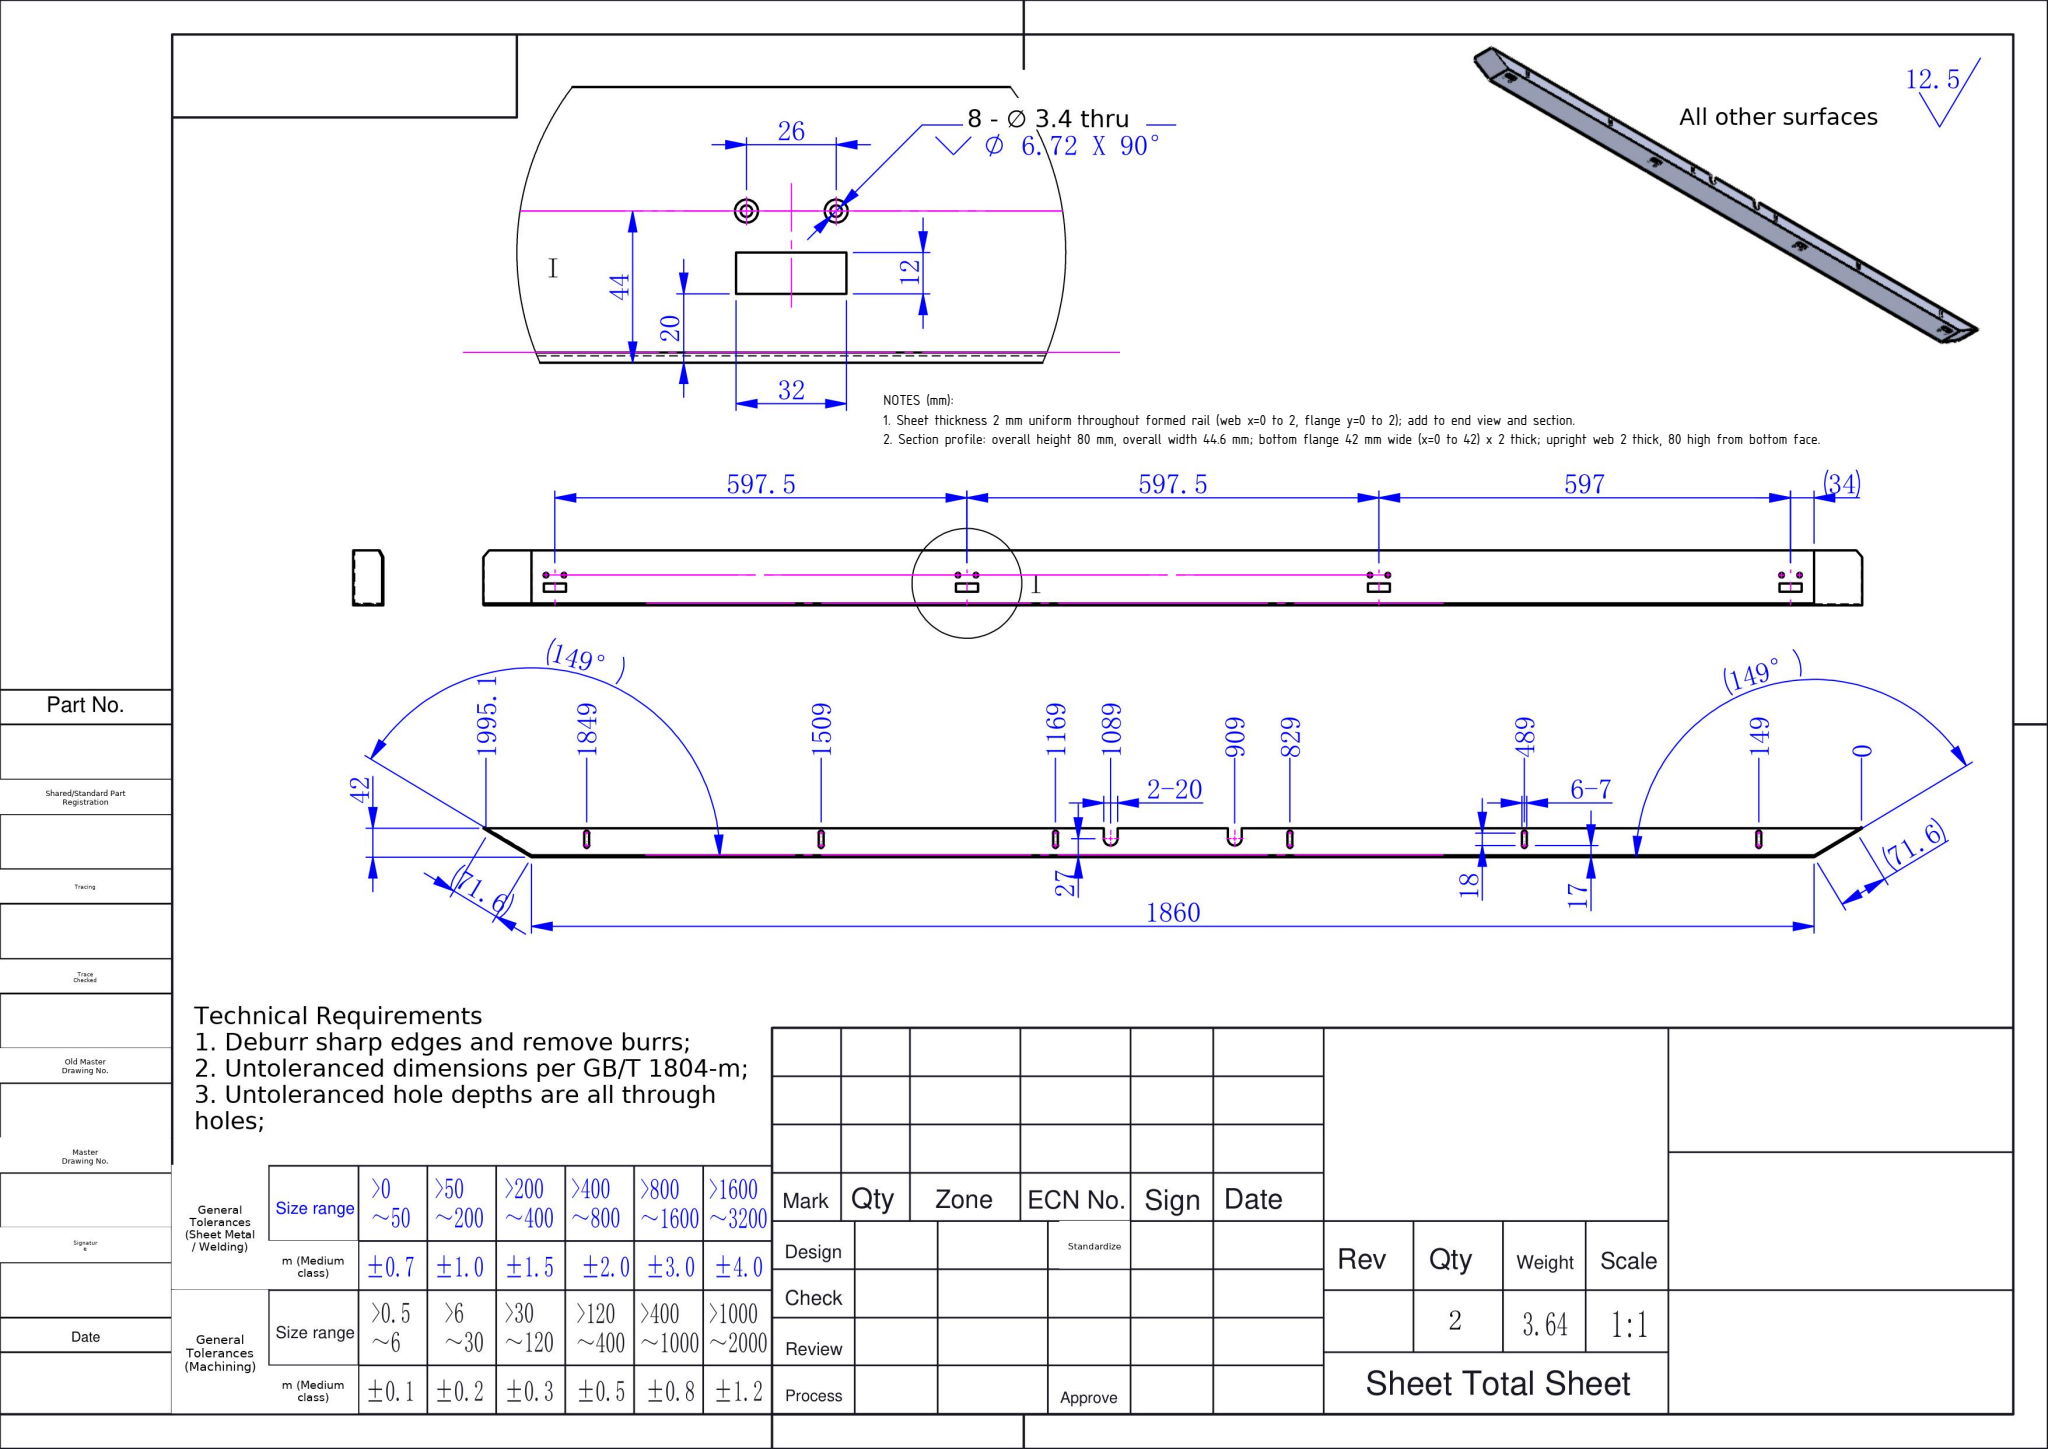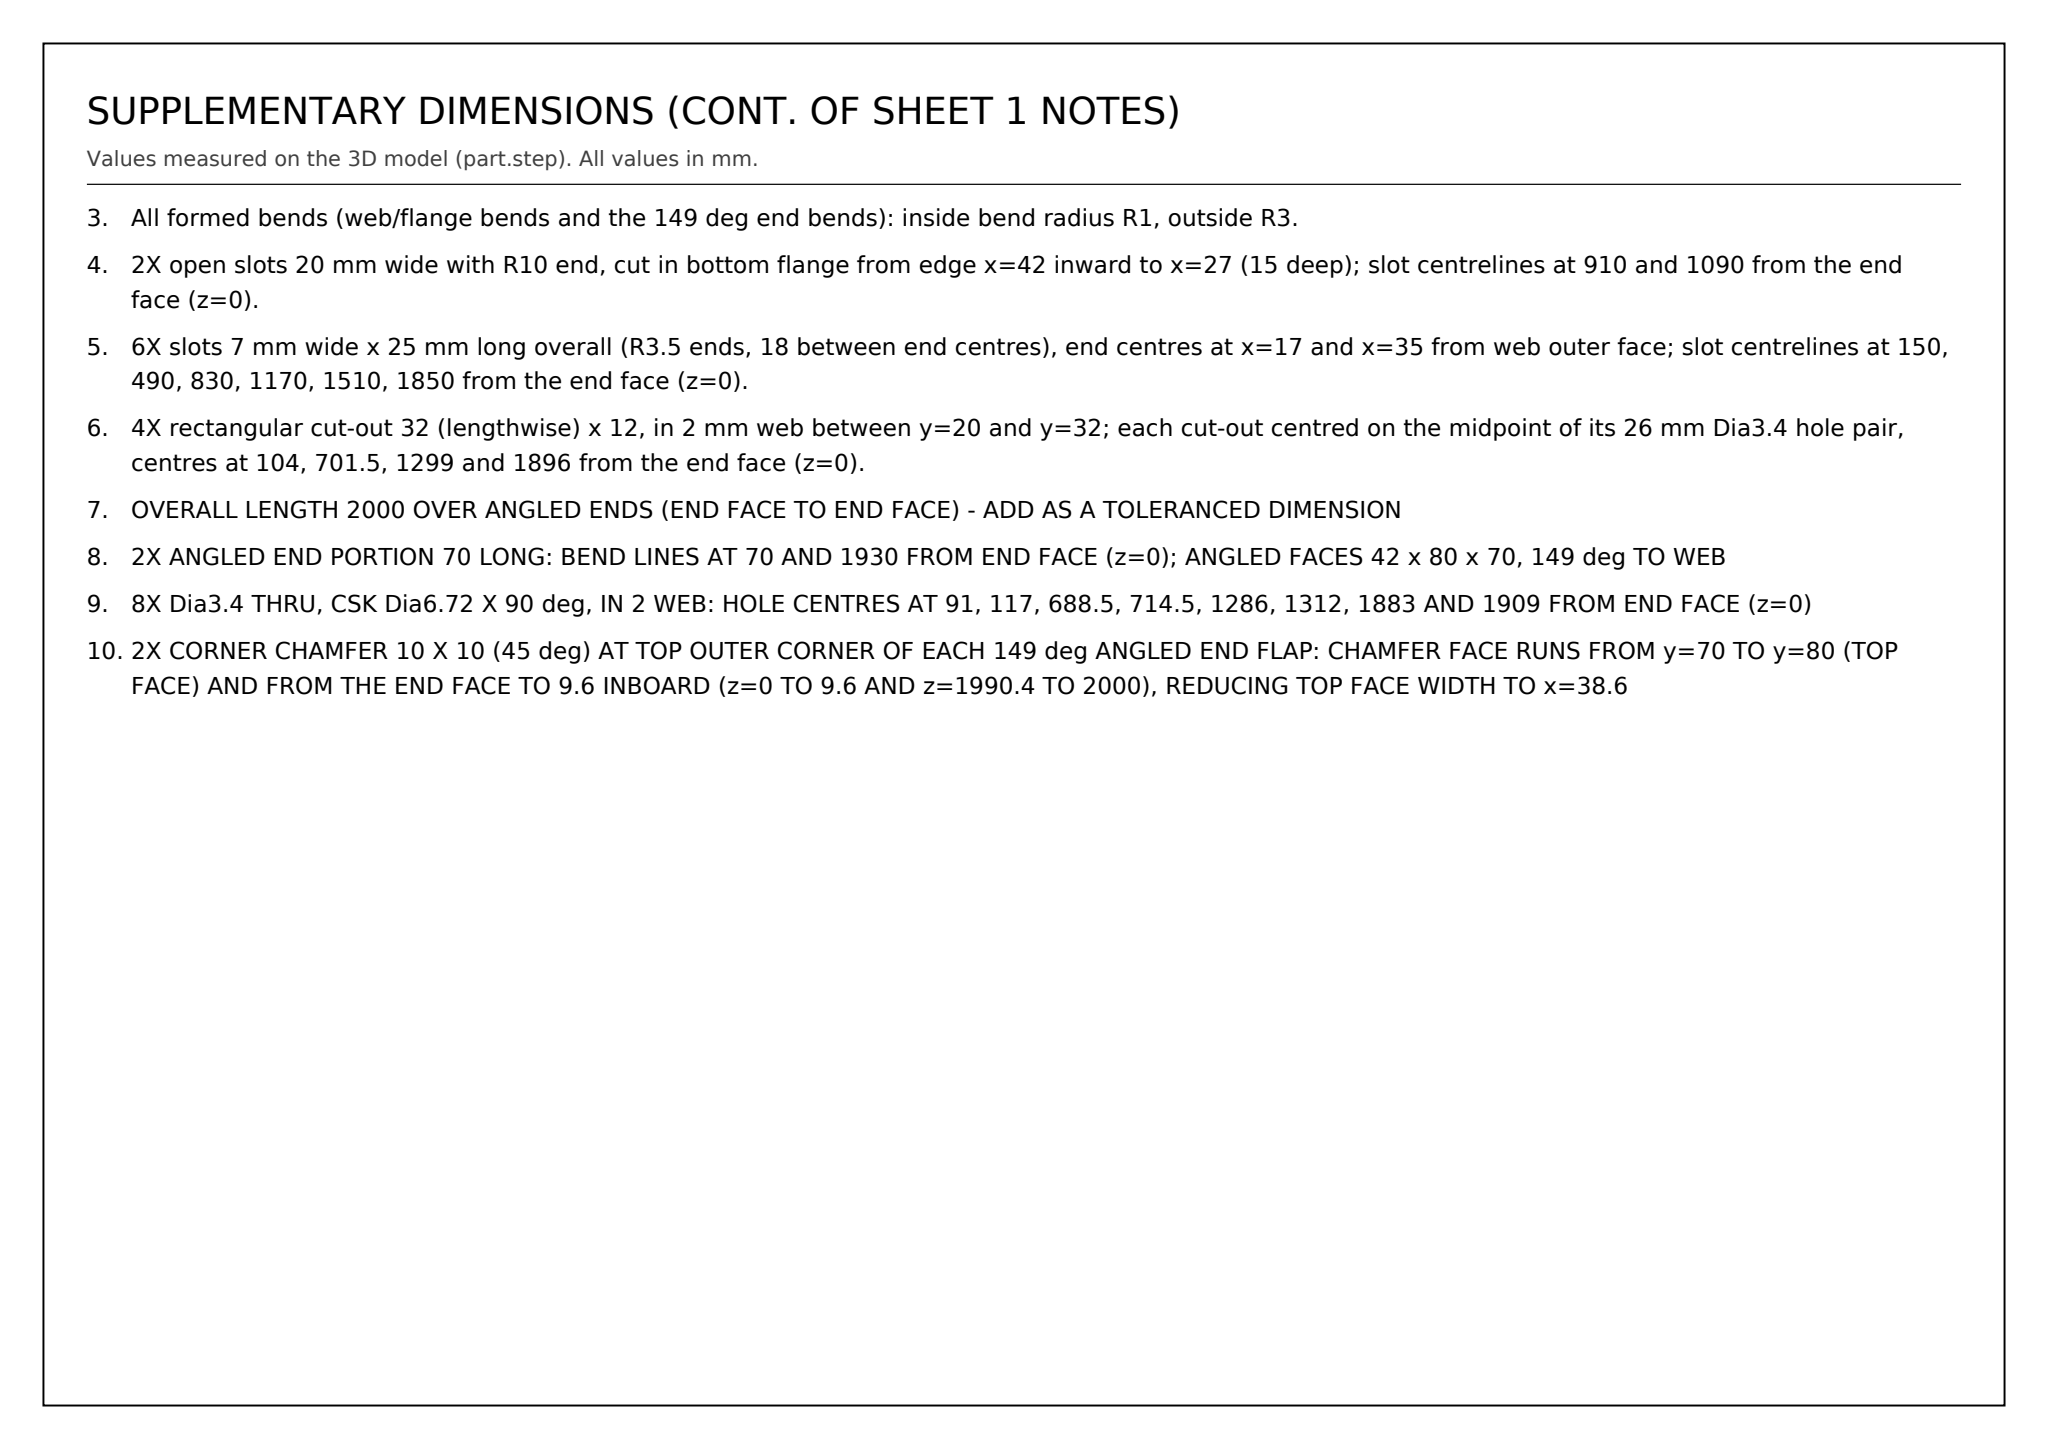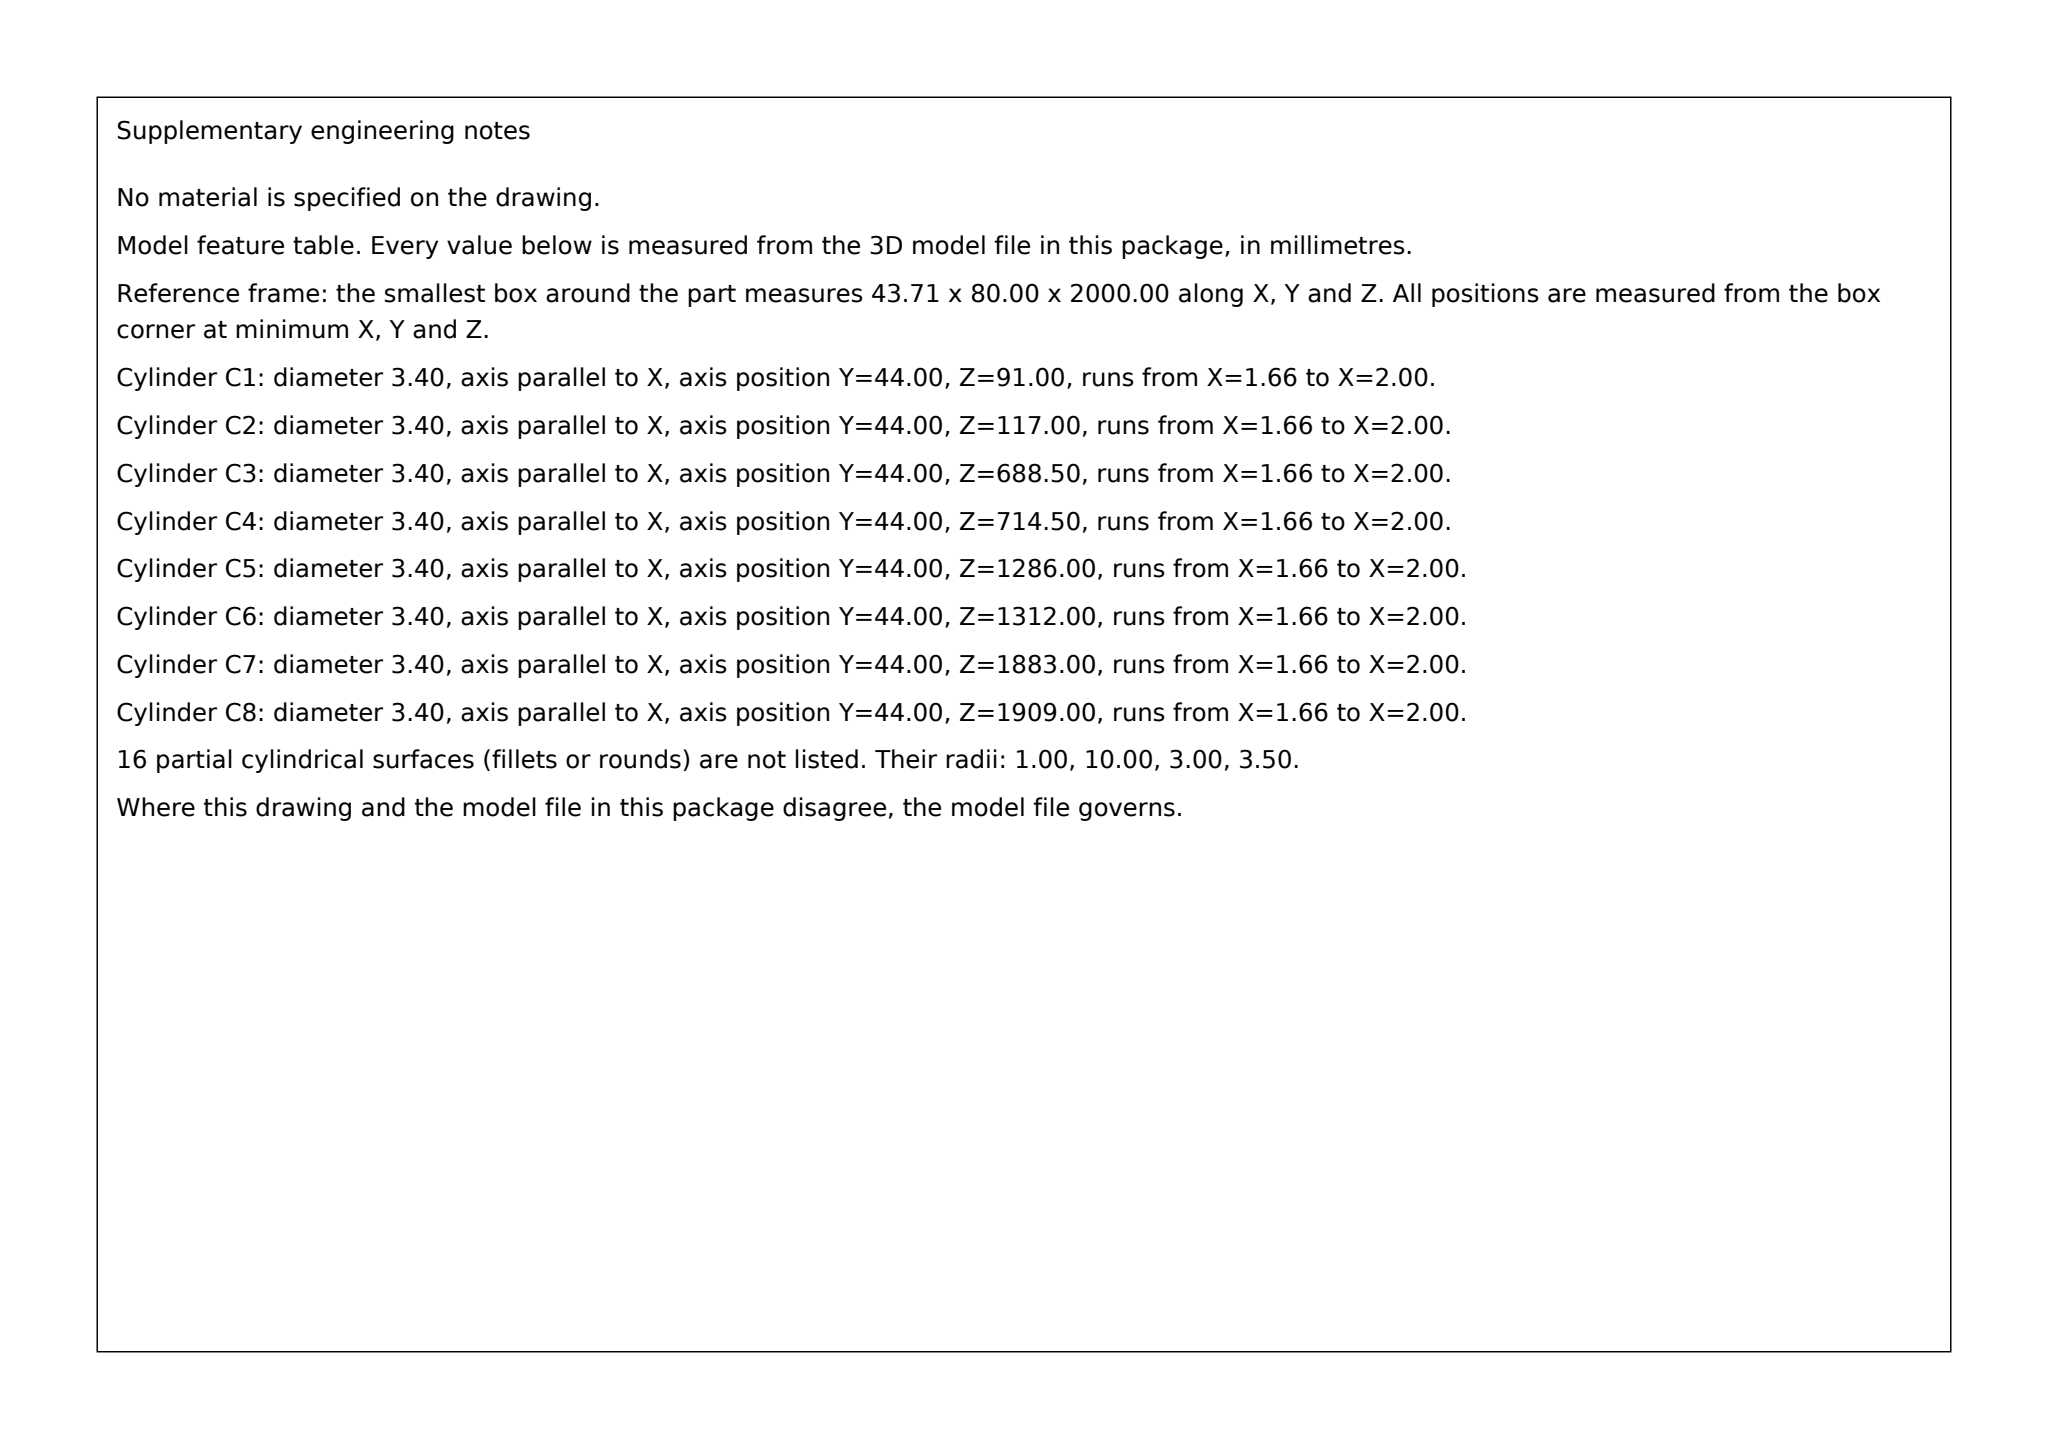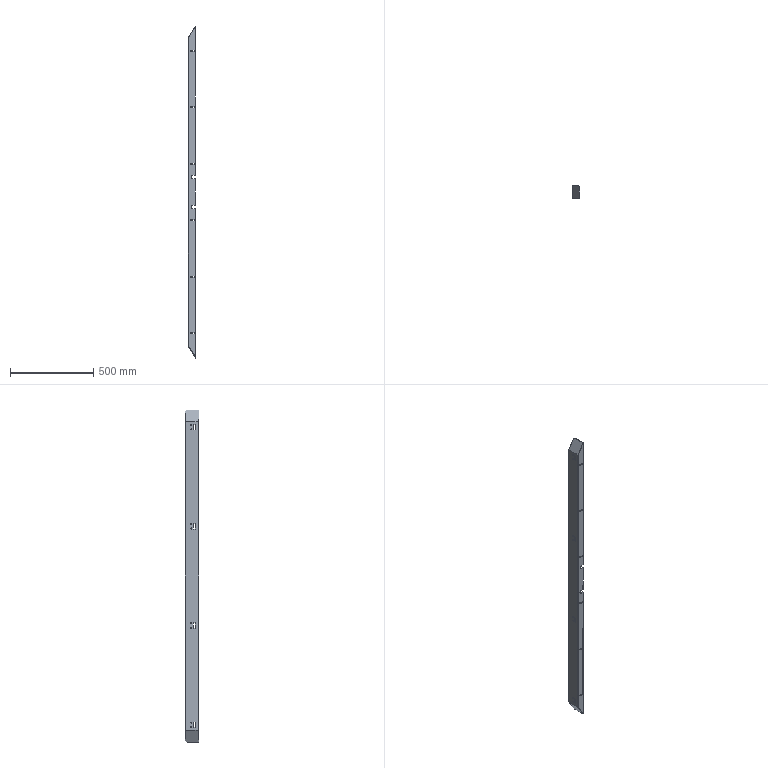Part | SolidWorks | mm | 1 solid | 101 faces | box 43.71 x 80 x 2000 mm | volume 466865 mm3 | plane 52 | cylinder 33 | cone 16 | commonest cylinder face diameters 3.4 x16 7 x12 6 x2 20 x2 2 x1
Drawing notes:
Sheet thickness 2 mm uniform throughout formed rail (web x=0 to 2, flange y=0 to 2); add to end view and section. | from the solid: axis_planes x normal at offset 0.0 and 2.0 (parallel faces 2 apart); y normal at offset 0.0 and 2.0
Section profile: overall height 80 mm, overall width 44.6 mm; bottom flange 42 mm wide (x=0 to 42) x 2 thick; upright web 2 thick, 80 high from bottom face. | from the solid: bbox_xyz [44.572, 80.0, 2000.0]; plane x=0 extent y 3-80; plane x=42 extent y 0-2; plane y=80 extent x 0-38.6
All formed bends (web/flange bends and the 149 deg end bends): inside bend radius R1, outside R3. | from the solid: concave arc dia 2.0 axis z at (3.0,3.0) 90 deg; convex arcs dia 6.0 (axis z and inclined at 44.6,3.0) 90 deg
2X open slots 20 mm wide with R10 end, cut in bottom flange from edge x=42 inward to x=27 (15 deep); slot centrelines at 910 and 1090 from the end face (z=0). | from the solid: concave arcs dia 20.0 axis y at x=27, z=910 and z=1090, 180 deg; planes z=900/920 and z=1080/1100 extent x 27-42
6X slots 7 mm wide x 25 mm long overall (R3.5 ends, 18 between end centres), end centres at x=17 and x=35 from web outer face; slot centrelines at 150, 490, 830, 1170, 1510, 1850 from the end face (z=0). | from the solid: concave arcs dia 7.0 axis y at x=17 and x=35, z=150/490/830/1170/1510/1850; planes z=146.5/153.5 extent x 17-35
4X rectangular cut-out 32 (lengthwise) x 12, in 2 mm web between y=20 and y=32; each cut-out centred on the midpoint of its 26 mm Dia3.4 hole pair, centres at 104, 701.5, 1299 and 1896 from the end face (z=0). | from the solid: planes y=20 and y=32 extents z 88-120, 685.5-717.5, 1283-1315, 1880-1912; holes dia 3.4 at z=91/117, 688.5/714.5, 1286/1312, 1883/1909
OVERALL LENGTH 2000 OVER ANGLED ENDS (END FACE TO END FACE) - ADD AS A TOLERANCED DIMENSION | from the solid: bbox_xyz = [44.572, 80.0, 2000.0] (z extent 0 to 2000)
2X ANGLED END PORTION 70 LONG: BEND LINES AT 70 AND 1930 FROM END FACE (z=0); ANGLED FACES 42 x 80 x 70, 149 deg TO WEB | from the solid: inclined_planes: bbox_from [0,0,1930] size [42,80,70] and [0,3,0] size [42,77,70]; plane x=0 extent z 70 to 1930
8X Dia3.4 THRU, CSK Dia6.72 X 90 deg, IN 2 WEB: HOLE CENTRES AT 91, 117, 688.5, 714.5, 1286, 1312, 1883 AND 1909 FROM END FACE (z=0) | from the solid: cylinders hole/bore dia 3.4 axis x at z = 91, 117, 688.5, 714.5, 1286, 1312, 1883, 1909 (y=44)
2X CORNER CHAMFER 10 X 10 (45 deg) AT TOP OUTER CORNER OF EACH 149 deg ANGLED END FLAP: CHAMFER FACE RUNS FROM y=70 TO y=80 (TOP FACE) AND FROM THE END FACE TO 9.6 INBOARD (z=0 TO 9.6 AND z=1990.4 TO 2000), REDUCING TOP FACE WIDTH TO x=38.6 | from the solid: inclined_planes: angle_to_xyz_axes [68.7,45.0,52.7], bbox_from [36.9,70.0,0.0] and [36.9,70.0,1990.4], size [6.9,10.0,9.6]; axis_plane y=80 extent x [0.0,38.6], z [8.6,1991.4]